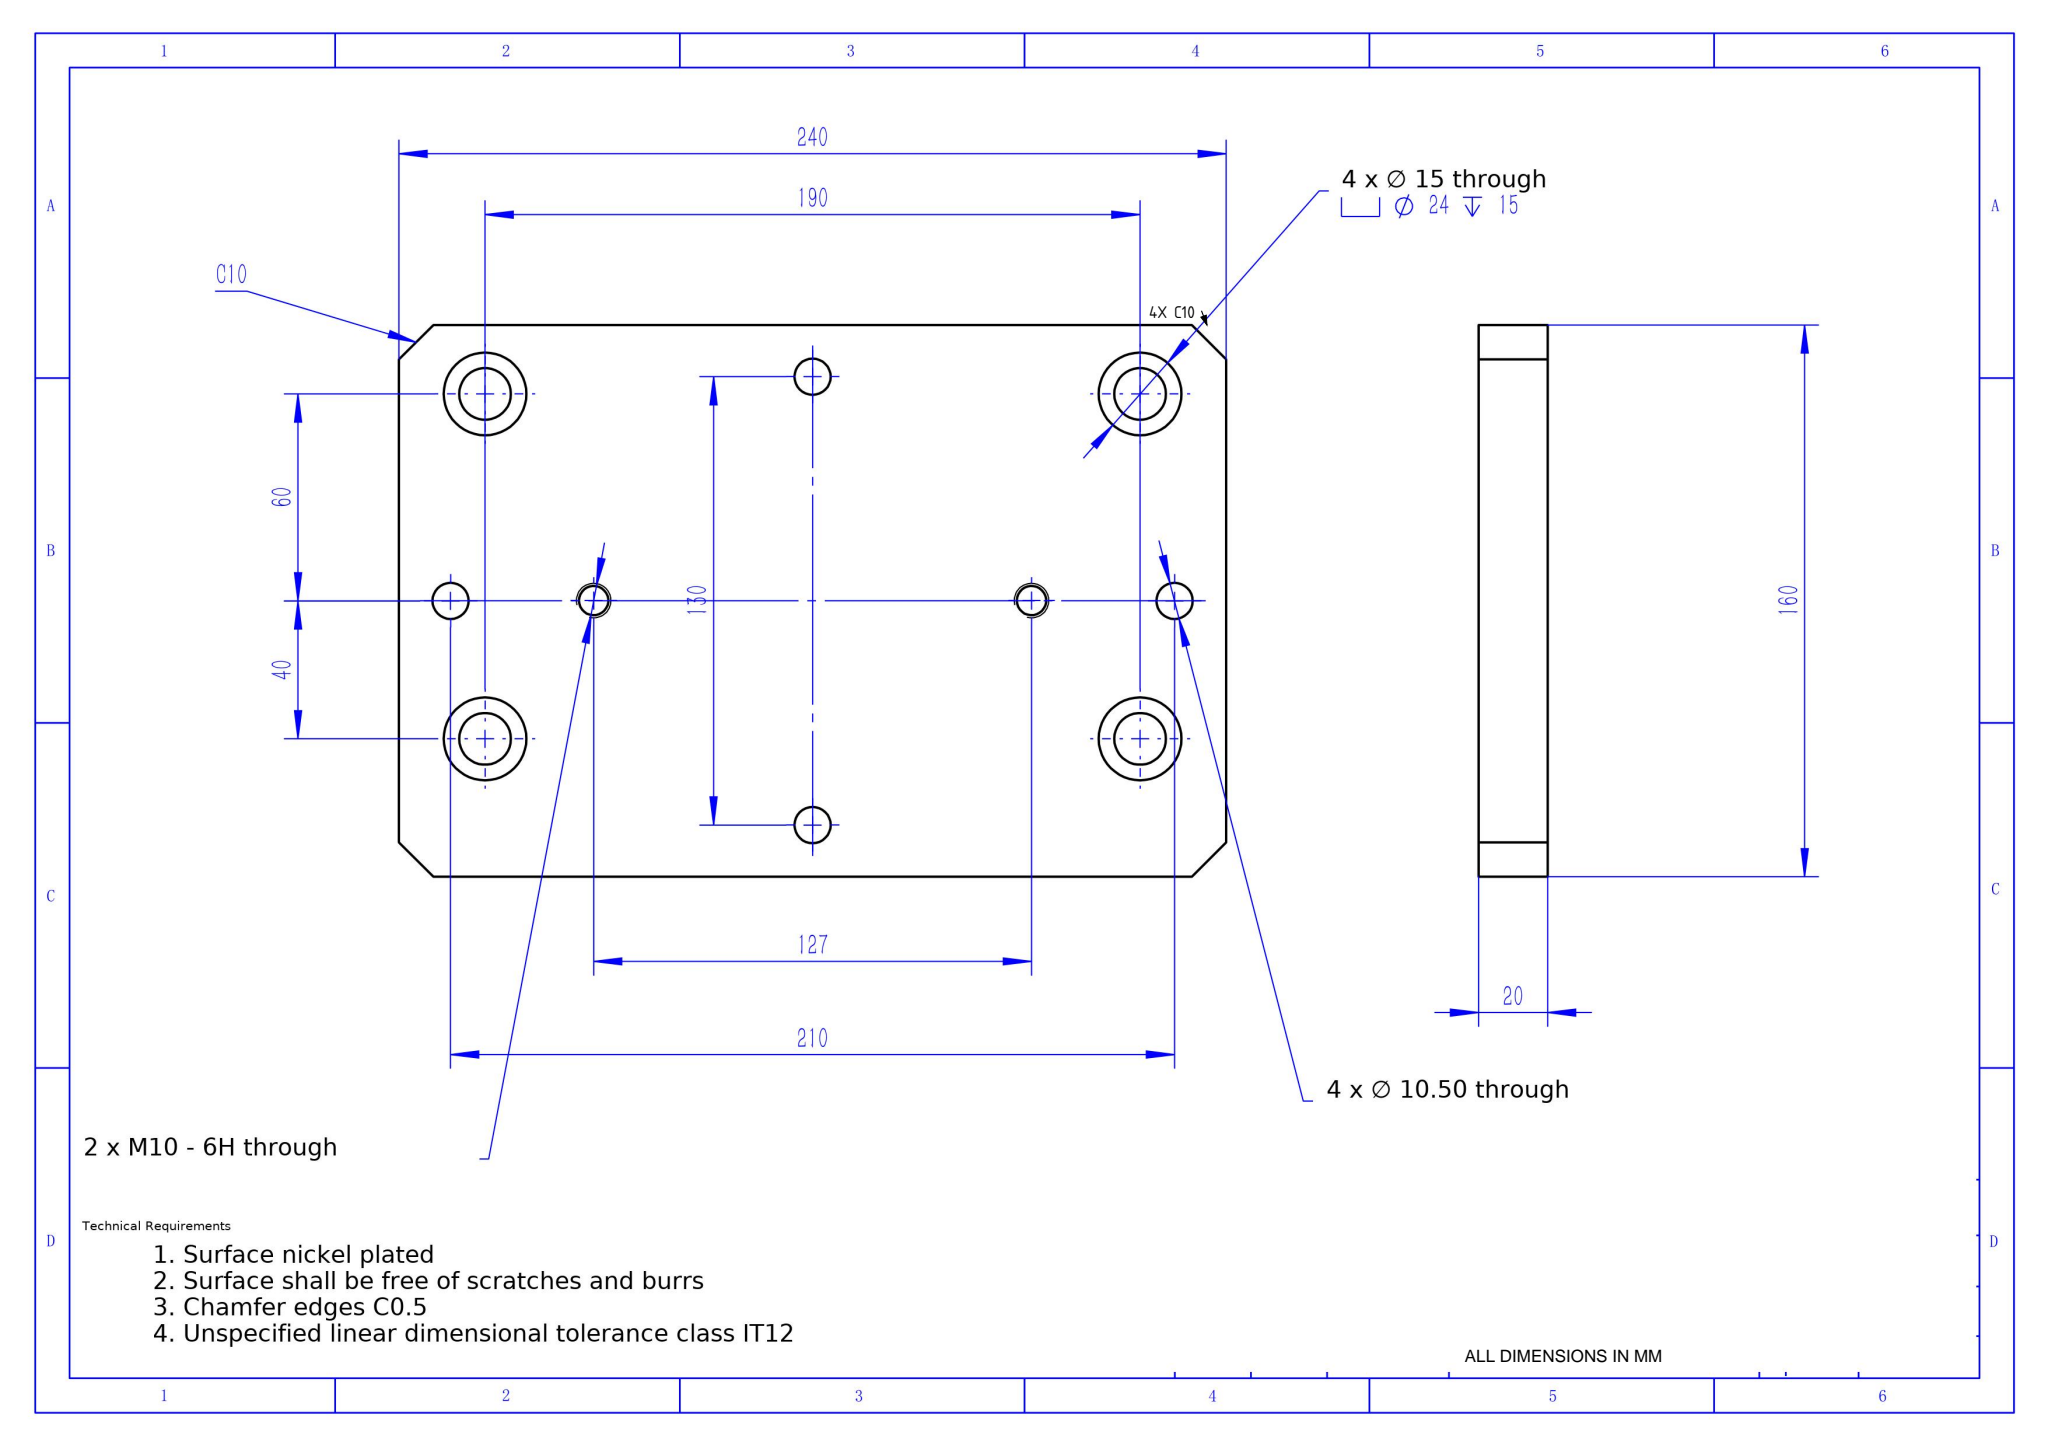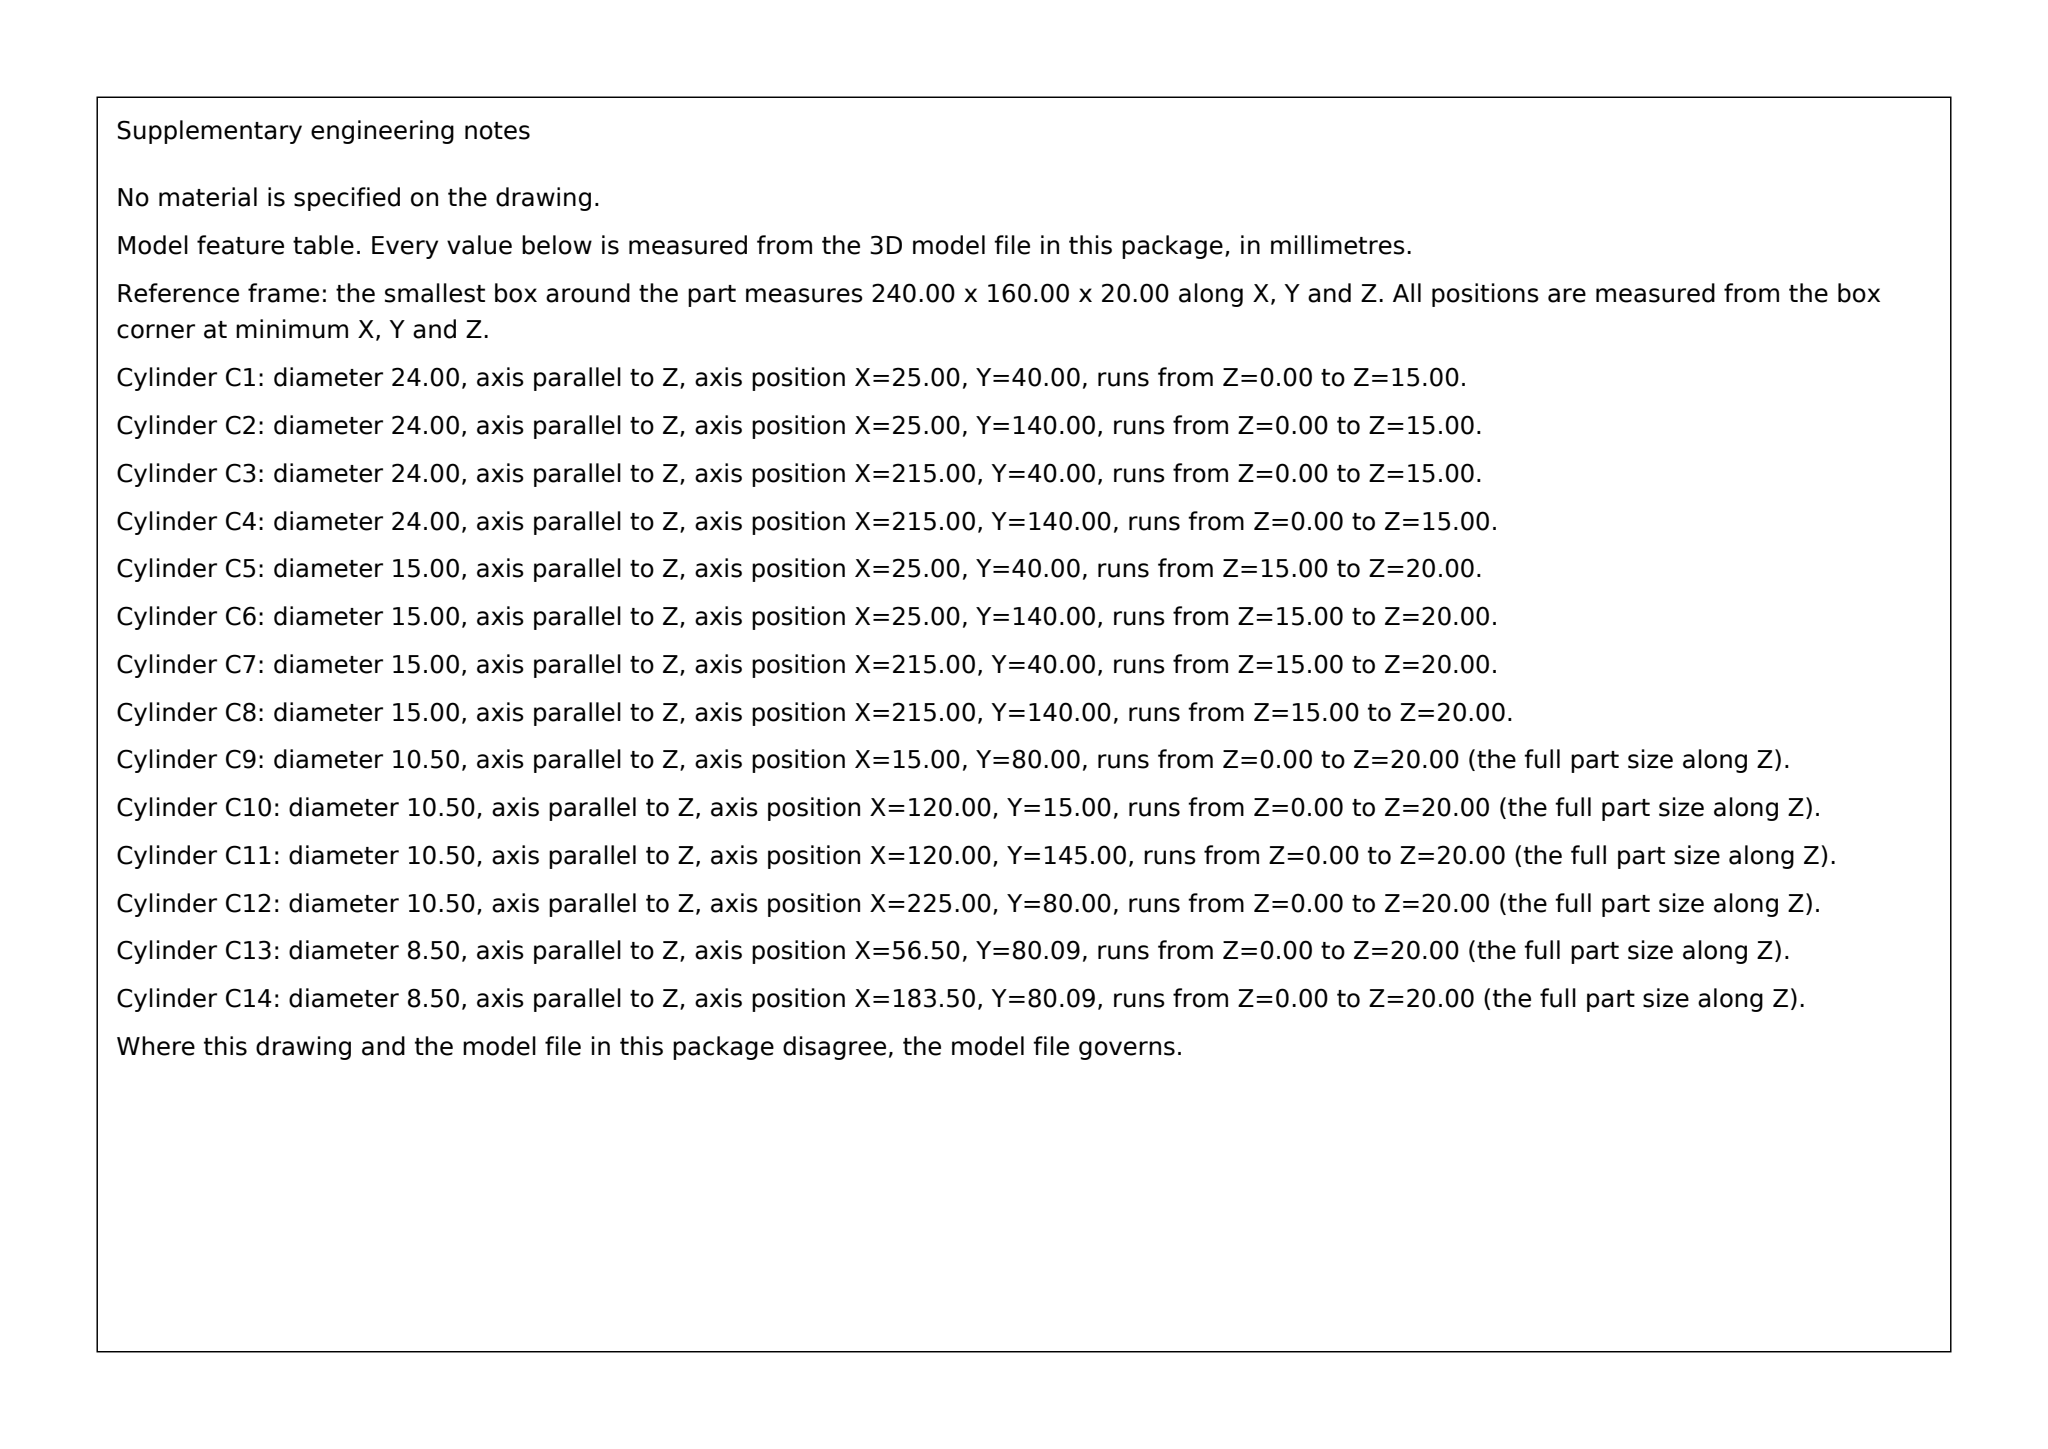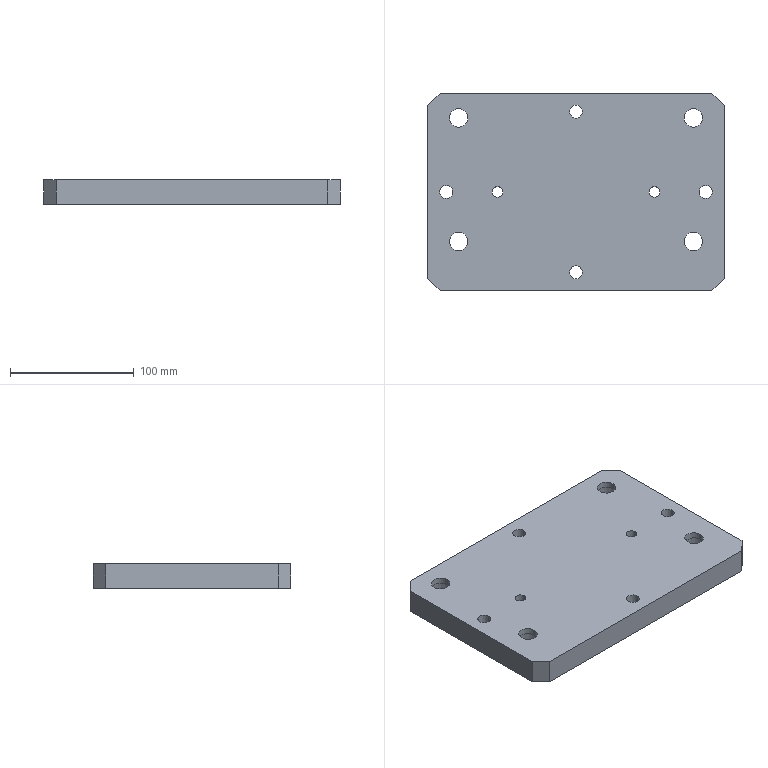Part | SolidWorks | mm | 1 solid | 42 faces | box 240 x 160 x 20 mm | volume 724125 mm3 | cylinder 28 | plane 14 | commonest cylinder face diameters 10.5 x8 24 x8 15 x8 8.5 x4
Drawing notes:
CORNER CHAMFERS C10 - 4 PLCS (TYP) | from the solid: 240x160 plate outline with 10x10 cut at all four corners (x0/x240, y0/y160)
build123d program:
from build123d import *

# Parameters (mm, degrees)
SKETCH1_W                                         = 240
SKETCH1_H                                         = 160
BOSS_EXTRUDE1_DEPTH                               = 20
HOLE_SIZE_ACCORDING_TO_TYPE_1_OF_HEXA_D           = 15
HOLE_SIZE_ACCORDING_TO_TYPE_1_OF_HEXA_CBORE_D     = 24
HOLE_SIZE_ACCORDING_TO_TYPE_1_OF_HEXA_CBORE_DEPTH = 15
CHAMFER1_SIZE                                     = 10
F_10_5_10_5_DIAMETER_HOLE1_D                      = 10.5
M10_TAPPED_HOLE1_D                                = 8.5


with BuildPart() as part:
    # Sketch1 → Boss-Extrude1 (new body)
    with BuildSketch(Plane.XY):
        with Locations((120, 80)):
            Rectangle(SKETCH1_W, SKETCH1_H)
    extrude(amount=BOSS_EXTRUDE1_DEPTH)

    # Hole Size _ according to_ type 1 of Hexa (through all)
    with Locations(Plane(origin=(0, 0, 0), x_dir=(-1, 0, 0), z_dir=(0, 0, -1))):
        with Locations((-215, 140), (-25, 140), (-25, 40), (-215, 40)):
            CounterBoreHole(HOLE_SIZE_ACCORDING_TO_TYPE_1_OF_HEXA_D / 2, HOLE_SIZE_ACCORDING_TO_TYPE_1_OF_HEXA_CBORE_D / 2, HOLE_SIZE_ACCORDING_TO_TYPE_1_OF_HEXA_CBORE_DEPTH)

    # Chamfer1
    chamfer1_edges = [part.edges().sort_by_distance(p)[0] for p in [
        (0, 160, 10),
        (240, 160, 10),
        (240, 0, 10),
        (0, 0, 10),
    ]]
    chamfer(chamfer1_edges, length=CHAMFER1_SIZE)

    # 10.5 _10.5_ Diameter Hole1 (through all)
    with Locations(Plane.XY.offset(20)):
        with Locations((15, 80), (225, 80), (120, 145), (120, 15)):
            Hole(F_10_5_10_5_DIAMETER_HOLE1_D / 2)

    # M10 Tapped Hole1 (through all)
    with Locations(Plane.XY.offset(20)):
        with Locations((56.5, 80.088), (183.5, 80.088)):
            Hole(M10_TAPPED_HOLE1_D / 2)


solid = part.part